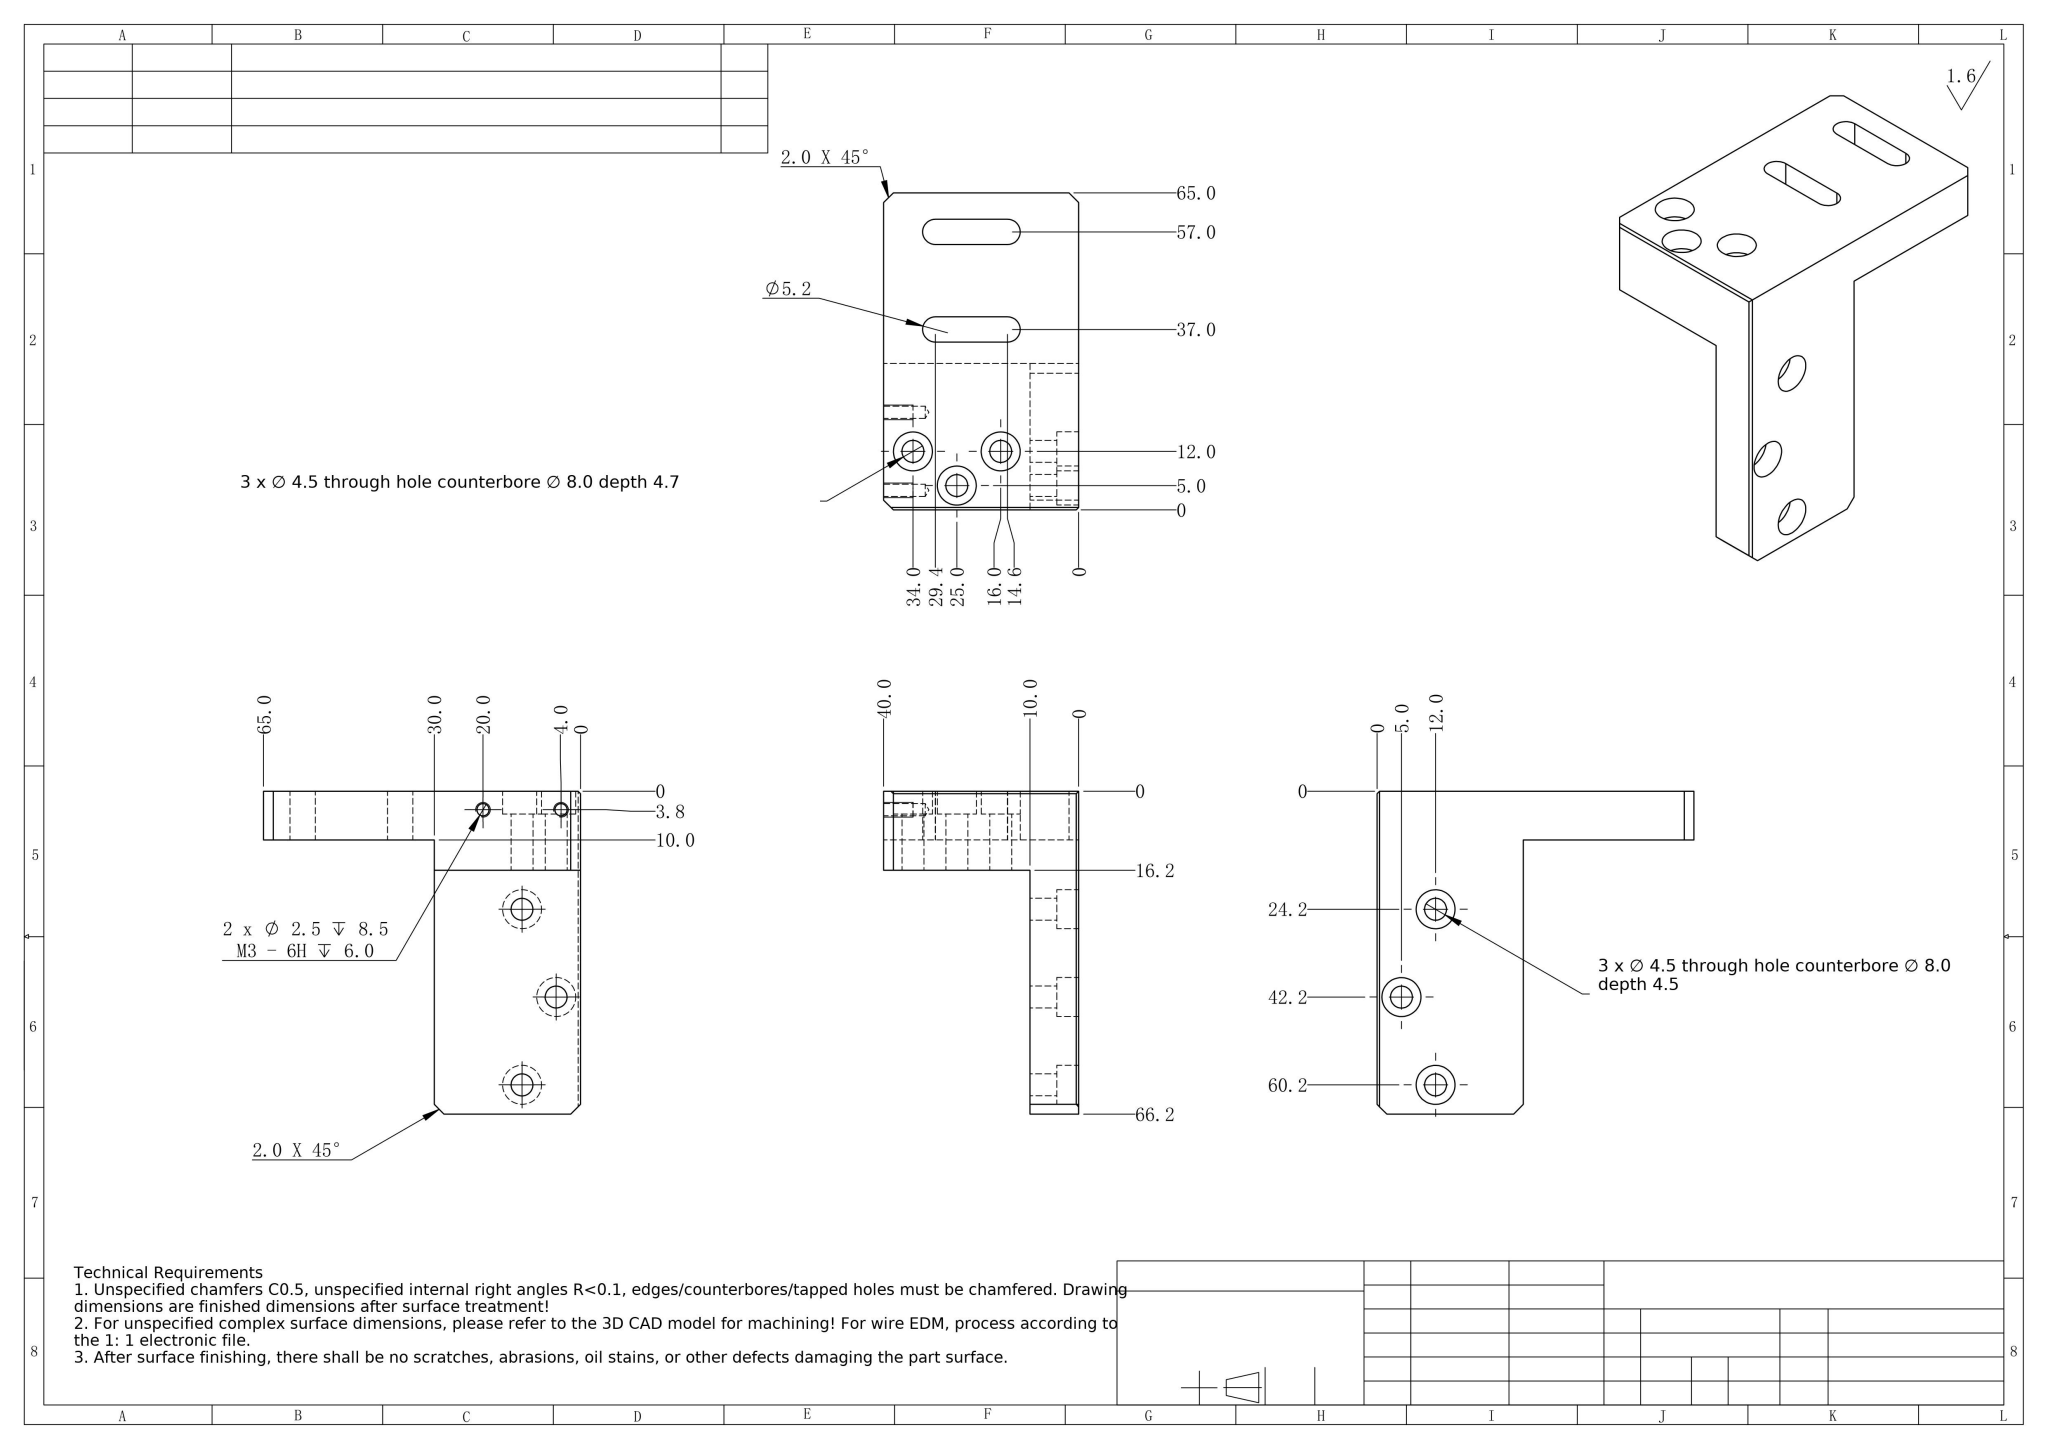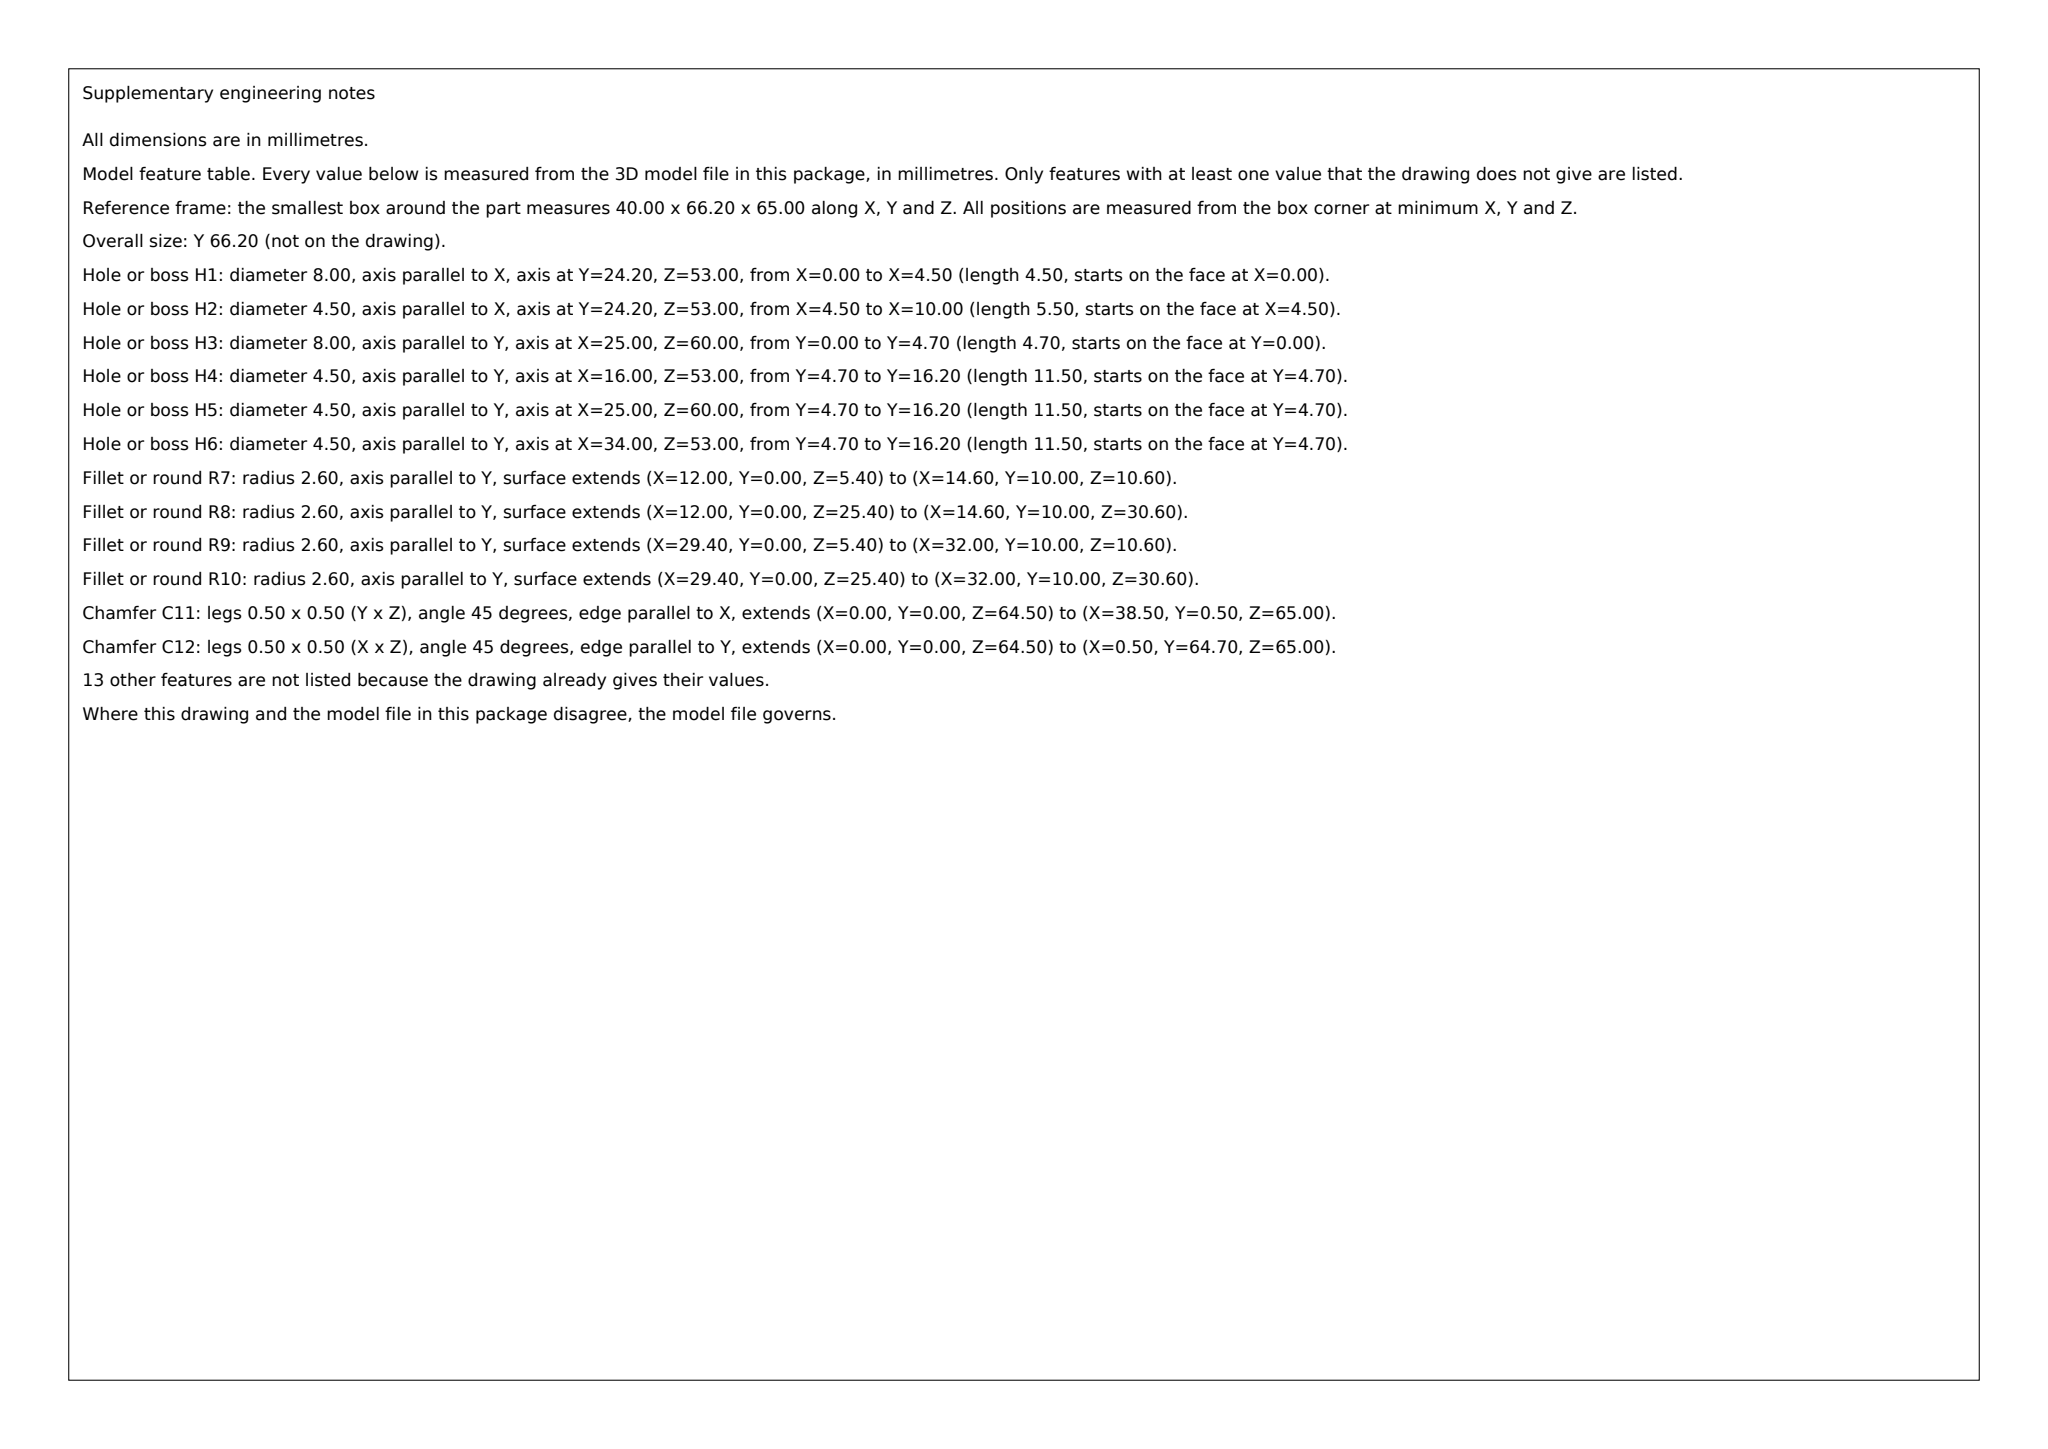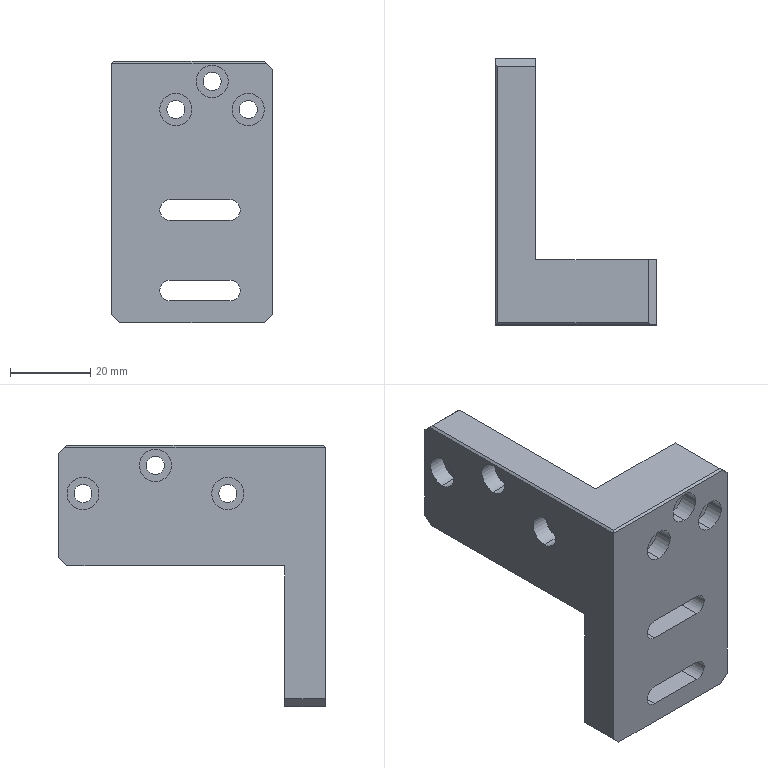Part | SolidWorks | mm | 1 solid | 63 faces | box 40 x 66.2 x 65 mm | volume 44067 mm3 | cylinder 32 | plane 27 | cone 4 | commonest cylinder face diameters 8 x12 4.5 x12 2.5 x4 5.2 x4